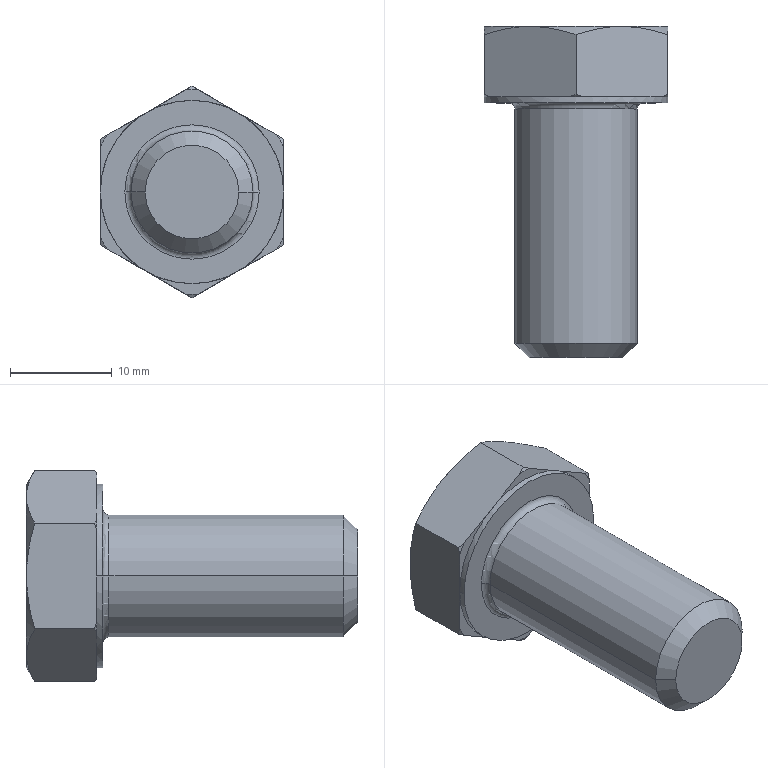Component | SolidWorks | GB_T5781-2000HexHeadBoltFullThreadCM12x25-2 | 1 solid | 35 faces | box 18 x 32.5 x 20.78 mm | volume 4879 mm3 | plane 15 | cone 14 | cylinder 4 | torus 2 | commonest cylinder face diameters 12 x2 18 x2 | material 3.6 Grade
STEP:
#1=CARTESIAN_POINT('',(0.5272,1.866,-3.022));
#2=VERTEX_POINT('',#1);
#3=CARTESIAN_POINT('',(0.05474,1.866,-3.022));
#4=VERTEX_POINT('',#3);
#5=CARTESIAN_POINT('',(0.291,1.866,-3.022));
#6=DIRECTION('',(0.,-1.,0.));
#7=DIRECTION('',(-1.,0.,0.));
#8=AXIS2_PLACEMENT_3D('',#5,#6,#7);
#9=CIRCLE('',#8,0.2362);
#10=EDGE_CURVE('',#2,#4,#9,.T.);
#11=ORIENTED_EDGE('',*,*,#10,.F.);
#12=CARTESIAN_POINT('',(0.5508,1.89,-3.022));
#13=VERTEX_POINT('',#12);
#14=CARTESIAN_POINT('',(0.5508,1.866,-3.022));
#15=DIRECTION('',(-0.,-0.,-1.));
#16=DIRECTION('',(-1.,0.,0.));
#17=AXIS2_PLACEMENT_3D('',#14,#15,#16);
#18=CIRCLE('',#17,0.02362);
#19=EDGE_CURVE('',#2,#13,#18,.T.);
#20=ORIENTED_EDGE('',*,*,#19,.T.);
#21=CARTESIAN_POINT('',(0.03111,1.89,-3.022));
#22=VERTEX_POINT('',#21);
#23=CARTESIAN_POINT('',(0.291,1.89,-3.022));
#24=DIRECTION('',(-0.,1.,-0.));
#25=DIRECTION('',(-1.,0.,0.));
#26=AXIS2_PLACEMENT_3D('',#23,#24,#25);
#27=CIRCLE('',#26,0.2598);
#28=EDGE_CURVE('',#22,#13,#27,.T.);
#29=ORIENTED_EDGE('',*,*,#28,.F.);
#30=CARTESIAN_POINT('',(0.03111,1.866,-3.022));
#31=DIRECTION('',(0.,0.,1.));
#32=DIRECTION('',(1.,0.,0.));
#33=AXIS2_PLACEMENT_3D('',#30,#31,#32);
#34=CIRCLE('',#33,0.02362);
#35=EDGE_CURVE('',#4,#22,#34,.T.);
#36=ORIENTED_EDGE('',*,*,#35,.F.);
#37=EDGE_LOOP('',(#11,#20,#29,#36));
#38=FACE_OUTER_BOUND('',#37,.T.);
#39=CARTESIAN_POINT('',(0.291,1.866,-3.022));
#40=DIRECTION('',(0.,-1.,0.));
#41=DIRECTION('',(-1.,-0.,0.));
#42=AXIS2_PLACEMENT_3D('',#39,#40,#41);
#43=TOROIDAL_SURFACE('',#42,0.2598,0.02362);
#44=ADVANCED_FACE('',(#38),#43,.F.);
#45=CARTESIAN_POINT('',(0.1099,0.9055,-3.022));
#46=VERTEX_POINT('',#45);
#47=CARTESIAN_POINT('',(0.4721,0.9055,-3.022));
#48=VERTEX_POINT('',#47);
#49=CARTESIAN_POINT('',(0.291,0.9055,-3.022));
#50=DIRECTION('',(0.,-1.,0.));
#51=DIRECTION('',(1.,0.,-0.));
#52=AXIS2_PLACEMENT_3D('',#49,#50,#51);
#53=CIRCLE('',#52,0.1811);
#54=EDGE_CURVE('',#46,#48,#53,.T.);
#55=ORIENTED_EDGE('',*,*,#54,.F.);
#56=CARTESIAN_POINT('',(0.05474,0.9606,-3.022));
#57=VERTEX_POINT('',#56);
#58=CARTESIAN_POINT('',(0.05474,0.9606,-3.022));
#59=DIRECTION('',(-0.7071,0.7071,0.));
#60=VECTOR('',#59,39.37);
#61=LINE('',#58,#60);
#62=EDGE_CURVE('',#46,#57,#61,.T.);
#63=ORIENTED_EDGE('',*,*,#62,.T.);
#64=CARTESIAN_POINT('',(0.5272,0.9606,-3.022));
#65=VERTEX_POINT('',#64);
#66=CARTESIAN_POINT('',(0.291,0.9606,-3.022));
#67=DIRECTION('',(-0.,1.,-0.));
#68=DIRECTION('',(1.,0.,-0.));
#69=AXIS2_PLACEMENT_3D('',#66,#67,#68);
#70=CIRCLE('',#69,0.2362);
#71=EDGE_CURVE('',#65,#57,#70,.T.);
#72=ORIENTED_EDGE('',*,*,#71,.F.);
#73=CARTESIAN_POINT('',(0.5272,0.9606,-3.022));
#74=DIRECTION('',(0.7071,0.7071,-0.));
#75=VECTOR('',#74,39.37);
#76=LINE('',#73,#75);
#77=EDGE_CURVE('',#48,#65,#76,.T.);
#78=ORIENTED_EDGE('',*,*,#77,.F.);
#79=EDGE_LOOP('',(#55,#63,#72,#78));
#80=FACE_OUTER_BOUND('',#79,.T.);
#81=CARTESIAN_POINT('',(0.291,0.9606,-3.022));
#82=DIRECTION('',(-0.,1.,-0.));
#83=DIRECTION('',(1.,0.,-0.));
#84=AXIS2_PLACEMENT_3D('',#81,#82,#83);
#85=CONICAL_SURFACE('',#84,0.2362,0.7854);
#86=ADVANCED_FACE('',(#80),#85,.T.);
#87=ORIENTED_EDGE('',*,*,#71,.T.);
#88=CARTESIAN_POINT('',(0.05474,2.185,-3.022));
#89=DIRECTION('',(-0.,1.,-0.));
#90=VECTOR('',#89,39.37);
#91=LINE('',#88,#90);
#92=EDGE_CURVE('',#57,#4,#91,.T.);
#93=ORIENTED_EDGE('',*,*,#92,.T.);
#94=CARTESIAN_POINT('',(0.291,1.866,-3.022));
#95=DIRECTION('',(0.,-1.,0.));
#96=DIRECTION('',(-1.,0.,0.));
#97=AXIS2_PLACEMENT_3D('',#94,#95,#96);
#98=CIRCLE('',#97,0.2362);
#99=EDGE_CURVE('',#4,#2,#98,.T.);
#100=ORIENTED_EDGE('',*,*,#99,.T.);
#101=CARTESIAN_POINT('',(0.5272,2.185,-3.022));
#102=DIRECTION('',(-0.,1.,-0.));
#103=VECTOR('',#102,39.37);
#104=LINE('',#101,#103);
#105=EDGE_CURVE('',#65,#2,#104,.T.);
#106=ORIENTED_EDGE('',*,*,#105,.F.);
#107=EDGE_LOOP('',(#87,#93,#100,#106));
#108=FACE_OUTER_BOUND('',#107,.T.);
#109=CARTESIAN_POINT('',(0.291,2.185,-3.022));
#110=DIRECTION('',(-0.,1.,-0.));
#111=DIRECTION('',(1.,0.,-0.));
#112=AXIS2_PLACEMENT_3D('',#109,#110,#111);
#113=CYLINDRICAL_SURFACE('',#112,0.2362);
#114=ADVANCED_FACE('',(#108),#113,.T.);
#115=CARTESIAN_POINT('',(-0.06337,1.89,-3.022));
#116=VERTEX_POINT('',#115);
#117=CARTESIAN_POINT('',(0.6453,1.89,-3.022));
#118=VERTEX_POINT('',#117);
#119=CARTESIAN_POINT('',(0.291,1.89,-3.022));
#120=DIRECTION('',(0.,-1.,0.));
#121=DIRECTION('',(-1.,0.,0.));
#122=AXIS2_PLACEMENT_3D('',#119,#120,#121);
#123=CIRCLE('',#122,0.3543);
#124=EDGE_CURVE('',#116,#118,#123,.T.);
#125=ORIENTED_EDGE('',*,*,#124,.F.);
#126=CARTESIAN_POINT('',(-0.06337,1.913,-3.022));
#127=VERTEX_POINT('',#126);
#128=CARTESIAN_POINT('',(-0.06337,2.185,-3.022));
#129=DIRECTION('',(-0.,1.,-0.));
#130=VECTOR('',#129,39.37);
#131=LINE('',#128,#130);
#132=EDGE_CURVE('',#116,#127,#131,.T.);
#133=ORIENTED_EDGE('',*,*,#132,.T.);
#134=CARTESIAN_POINT('',(0.1138,1.913,-3.329));
#135=VERTEX_POINT('',#134);
#136=CARTESIAN_POINT('',(0.291,1.913,-3.022));
#137=DIRECTION('',(-0.,1.,-0.));
#138=DIRECTION('',(1.,0.,-0.));
#139=AXIS2_PLACEMENT_3D('',#136,#137,#138);
#140=CIRCLE('',#139,0.3543);
#141=EDGE_CURVE('',#135,#127,#140,.T.);
#142=ORIENTED_EDGE('',*,*,#141,.F.);
#143=CARTESIAN_POINT('',(0.4681,1.913,-3.329));
#144=VERTEX_POINT('',#143);
#145=CARTESIAN_POINT('',(0.291,1.913,-3.022));
#146=DIRECTION('',(-0.,1.,-0.));
#147=DIRECTION('',(1.,0.,-0.));
#148=AXIS2_PLACEMENT_3D('',#145,#146,#147);
#149=CIRCLE('',#148,0.3543);
#150=EDGE_CURVE('',#144,#135,#149,.T.);
#151=ORIENTED_EDGE('',*,*,#150,.F.);
#152=CARTESIAN_POINT('',(0.6453,1.913,-3.022));
#153=VERTEX_POINT('',#152);
#154=CARTESIAN_POINT('',(0.291,1.913,-3.022));
#155=DIRECTION('',(-0.,1.,-0.));
#156=DIRECTION('',(1.,0.,-0.));
#157=AXIS2_PLACEMENT_3D('',#154,#155,#156);
#158=CIRCLE('',#157,0.3543);
#159=EDGE_CURVE('',#153,#144,#158,.T.);
#160=ORIENTED_EDGE('',*,*,#159,.F.);
#161=CARTESIAN_POINT('',(0.6453,2.185,-3.022));
#162=DIRECTION('',(-0.,1.,-0.));
#163=VECTOR('',#162,39.37);
#164=LINE('',#161,#163);
#165=EDGE_CURVE('',#118,#153,#164,.T.);
#166=ORIENTED_EDGE('',*,*,#165,.F.);
#167=EDGE_LOOP('',(#125,#133,#142,#151,#160,#166));
#168=FACE_OUTER_BOUND('',#167,.T.);
#169=CARTESIAN_POINT('',(0.291,2.185,-3.022));
#170=DIRECTION('',(-0.,1.,-0.));
#171=DIRECTION('',(1.,0.,-0.));
#172=AXIS2_PLACEMENT_3D('',#169,#170,#171);
#173=CYLINDRICAL_SURFACE('',#172,0.3543);
#174=ADVANCED_FACE('',(#168),#173,.T.);
#175=CARTESIAN_POINT('',(-0.03787,1.913,-3.241));
#176=VERTEX_POINT('',#175);
#177=CARTESIAN_POINT('',(-0.06337,1.913,-3.227));
#178=DIRECTION('',(0.866,0.,-0.5));
#179=VECTOR('',#178,39.37);
#180=LINE('',#177,#179);
#181=EDGE_CURVE('',#176,#135,#180,.T.);
#182=ORIENTED_EDGE('',*,*,#181,.F.);
#183=CARTESIAN_POINT('',(-0.06337,1.921,-3.227));
#184=VERTEX_POINT('',#183);
#185=CARTESIAN_POINT('',(-0.06337,1.921,-3.227));
#186=CARTESIAN_POINT('',(-0.05489,1.919,-3.232));
#187=CARTESIAN_POINT('',(-0.04639,1.916,-3.237));
#188=CARTESIAN_POINT('',(-0.03787,1.913,-3.241));
#189=B_SPLINE_CURVE_WITH_KNOTS('',3,(#185,#186,#187,#188),.UNSPECIFIED.,.F.,.F.,(4,4),(0.00000024,0.0007696),.UNSPECIFIED.);
#190=EDGE_CURVE('',#184,#176,#189,.T.);
#191=ORIENTED_EDGE('',*,*,#190,.F.);
#192=CARTESIAN_POINT('',(-0.06337,2.153,-3.227));
#193=VERTEX_POINT('',#192);
#194=CARTESIAN_POINT('',(-0.06337,1.89,-3.227));
#195=DIRECTION('',(-0.,1.,-0.));
#196=VECTOR('',#195,39.37);
#197=LINE('',#194,#196);
#198=EDGE_CURVE('',#184,#193,#197,.T.);
#199=ORIENTED_EDGE('',*,*,#198,.T.);
#200=CARTESIAN_POINT('',(0.1138,2.185,-3.329));
#201=VERTEX_POINT('',#200);
#202=CARTESIAN_POINT('',(0.1138,2.185,-3.329));
#203=CARTESIAN_POINT('',(0.09876,2.185,-3.32));
#204=CARTESIAN_POINT('',(0.08365,2.184,-3.312));
#205=CARTESIAN_POINT('',(0.05378,2.181,-3.294));
#206=CARTESIAN_POINT('',(0.03894,2.179,-3.286));
#207=CARTESIAN_POINT('',(-0.005313,2.171,-3.26));
#208=CARTESIAN_POINT('',(-0.03446,2.163,-3.243));
#209=CARTESIAN_POINT('',(-0.06337,2.153,-3.227));
#210=B_SPLINE_CURVE_WITH_KNOTS('',3,(#202,#203,#204,#205,#206,#207,#208,#209),.UNSPECIFIED.,.F.,.F.,(4,2,2,4),(0.005258,0.006567,0.007877,0.0105),.UNSPECIFIED.);
#211=EDGE_CURVE('',#201,#193,#210,.T.);
#212=ORIENTED_EDGE('',*,*,#211,.F.);
#213=CARTESIAN_POINT('',(0.291,2.153,-3.431));
#214=VERTEX_POINT('',#213);
#215=CARTESIAN_POINT('',(0.291,2.153,-3.431));
#216=CARTESIAN_POINT('',(0.262,2.163,-3.415));
#217=CARTESIAN_POINT('',(0.2328,2.171,-3.398));
#218=CARTESIAN_POINT('',(0.1738,2.182,-3.364));
#219=CARTESIAN_POINT('',(0.144,2.185,-3.346));
#220=CARTESIAN_POINT('',(0.1138,2.185,-3.329));
#221=B_SPLINE_CURVE_WITH_KNOTS('',3,(#215,#216,#217,#218,#219,#220),.UNSPECIFIED.,.F.,.F.,(4,2,4),(0.00000024,0.002629,0.005258),.UNSPECIFIED.);
#222=EDGE_CURVE('',#214,#201,#221,.T.);
#223=ORIENTED_EDGE('',*,*,#222,.F.);
#224=CARTESIAN_POINT('',(0.291,1.921,-3.431));
#225=VERTEX_POINT('',#224);
#226=CARTESIAN_POINT('',(0.291,1.89,-3.431));
#227=DIRECTION('',(-0.,1.,-0.));
#228=VECTOR('',#227,39.37);
#229=LINE('',#226,#228);
#230=EDGE_CURVE('',#225,#214,#229,.T.);
#231=ORIENTED_EDGE('',*,*,#230,.F.);
#232=CARTESIAN_POINT('',(0.2655,1.913,-3.417));
#233=VERTEX_POINT('',#232);
#234=CARTESIAN_POINT('',(0.2655,1.913,-3.417));
#235=CARTESIAN_POINT('',(0.274,1.916,-3.421));
#236=CARTESIAN_POINT('',(0.2825,1.919,-3.426));
#237=CARTESIAN_POINT('',(0.291,1.921,-3.431));
#238=B_SPLINE_CURVE_WITH_KNOTS('',3,(#234,#235,#236,#237),.UNSPECIFIED.,.F.,.F.,(4,4),(0.009728,0.0105),.UNSPECIFIED.);
#239=EDGE_CURVE('',#233,#225,#238,.T.);
#240=ORIENTED_EDGE('',*,*,#239,.F.);
#241=CARTESIAN_POINT('',(-0.06337,1.913,-3.227));
#242=DIRECTION('',(0.866,0.,-0.5));
#243=VECTOR('',#242,39.37);
#244=LINE('',#241,#243);
#245=EDGE_CURVE('',#135,#233,#244,.T.);
#246=ORIENTED_EDGE('',*,*,#245,.F.);
#247=EDGE_LOOP('',(#182,#191,#199,#212,#223,#231,#240,#246));
#248=FACE_OUTER_BOUND('',#247,.T.);
#249=CARTESIAN_POINT('',(-0.06337,1.89,-3.227));
#250=DIRECTION('',(0.5,0.,0.866));
#251=DIRECTION('',(-0.866,-0.,0.5));
#252=AXIS2_PLACEMENT_3D('',#249,#250,#251);
#253=PLANE('',#252);
#254=ADVANCED_FACE('',(#248),#253,.F.);
#255=CARTESIAN_POINT('',(0.3165,1.913,-3.417));
#256=VERTEX_POINT('',#255);
#257=CARTESIAN_POINT('',(0.291,1.913,-3.431));
#258=DIRECTION('',(0.866,0.,0.5));
#259=VECTOR('',#258,39.37);
#260=LINE('',#257,#259);
#261=EDGE_CURVE('',#256,#144,#260,.T.);
#262=ORIENTED_EDGE('',*,*,#261,.F.);
#263=CARTESIAN_POINT('',(0.291,1.921,-3.431));
#264=CARTESIAN_POINT('',(0.2994,1.919,-3.426));
#265=CARTESIAN_POINT('',(0.3079,1.916,-3.421));
#266=CARTESIAN_POINT('',(0.3165,1.913,-3.417));
#267=B_SPLINE_CURVE_WITH_KNOTS('',3,(#263,#264,#265,#266),.UNSPECIFIED.,.F.,.F.,(4,4),(0.00000024,0.0007696),.UNSPECIFIED.);
#268=EDGE_CURVE('',#225,#256,#267,.T.);
#269=ORIENTED_EDGE('',*,*,#268,.F.);
#270=ORIENTED_EDGE('',*,*,#230,.T.);
#271=CARTESIAN_POINT('',(0.4681,2.185,-3.329));
#272=VERTEX_POINT('',#271);
#273=CARTESIAN_POINT('',(0.4681,2.185,-3.329));
#274=CARTESIAN_POINT('',(0.4531,2.185,-3.338));
#275=CARTESIAN_POINT('',(0.438,2.184,-3.346));
#276=CARTESIAN_POINT('',(0.4081,2.181,-3.364));
#277=CARTESIAN_POINT('',(0.3933,2.179,-3.372));
#278=CARTESIAN_POINT('',(0.349,2.171,-3.398));
#279=CARTESIAN_POINT('',(0.3199,2.163,-3.415));
#280=CARTESIAN_POINT('',(0.291,2.153,-3.431));
#281=B_SPLINE_CURVE_WITH_KNOTS('',3,(#273,#274,#275,#276,#277,#278,#279,#280),.UNSPECIFIED.,.F.,.F.,(4,2,2,4),(0.005258,0.006567,0.007877,0.0105),.UNSPECIFIED.);
#282=EDGE_CURVE('',#272,#214,#281,.T.);
#283=ORIENTED_EDGE('',*,*,#282,.F.);
#284=CARTESIAN_POINT('',(0.6453,2.153,-3.227));
#285=VERTEX_POINT('',#284);
#286=CARTESIAN_POINT('',(0.6453,2.153,-3.227));
#287=CARTESIAN_POINT('',(0.6163,2.163,-3.243));
#288=CARTESIAN_POINT('',(0.5871,2.171,-3.26));
#289=CARTESIAN_POINT('',(0.5281,2.182,-3.294));
#290=CARTESIAN_POINT('',(0.4983,2.185,-3.312));
#291=CARTESIAN_POINT('',(0.4681,2.185,-3.329));
#292=B_SPLINE_CURVE_WITH_KNOTS('',3,(#286,#287,#288,#289,#290,#291),.UNSPECIFIED.,.F.,.F.,(4,2,4),(0.00000024,0.002629,0.005258),.UNSPECIFIED.);
#293=EDGE_CURVE('',#285,#272,#292,.T.);
#294=ORIENTED_EDGE('',*,*,#293,.F.);
#295=CARTESIAN_POINT('',(0.6453,1.921,-3.227));
#296=VERTEX_POINT('',#295);
#297=CARTESIAN_POINT('',(0.6453,1.89,-3.227));
#298=DIRECTION('',(-0.,1.,-0.));
#299=VECTOR('',#298,39.37);
#300=LINE('',#297,#299);
#301=EDGE_CURVE('',#296,#285,#300,.T.);
#302=ORIENTED_EDGE('',*,*,#301,.F.);
#303=CARTESIAN_POINT('',(0.6198,1.913,-3.241));
#304=VERTEX_POINT('',#303);
#305=CARTESIAN_POINT('',(0.6198,1.913,-3.241));
#306=CARTESIAN_POINT('',(0.6283,1.916,-3.237));
#307=CARTESIAN_POINT('',(0.6368,1.919,-3.232));
#308=CARTESIAN_POINT('',(0.6453,1.921,-3.227));
#309=B_SPLINE_CURVE_WITH_KNOTS('',3,(#305,#306,#307,#308),.UNSPECIFIED.,.F.,.F.,(4,4),(0.009728,0.0105),.UNSPECIFIED.);
#310=EDGE_CURVE('',#304,#296,#309,.T.);
#311=ORIENTED_EDGE('',*,*,#310,.F.);
#312=CARTESIAN_POINT('',(0.291,1.913,-3.431));
#313=DIRECTION('',(0.866,0.,0.5));
#314=VECTOR('',#313,39.37);
#315=LINE('',#312,#314);
#316=EDGE_CURVE('',#144,#304,#315,.T.);
#317=ORIENTED_EDGE('',*,*,#316,.F.);
#318=EDGE_LOOP('',(#262,#269,#270,#283,#294,#302,#311,#317));
#319=FACE_OUTER_BOUND('',#318,.T.);
#320=CARTESIAN_POINT('',(0.291,1.89,-3.431));
#321=DIRECTION('',(-0.5,0.,0.866));
#322=DIRECTION('',(-0.866,-0.,-0.5));
#323=AXIS2_PLACEMENT_3D('',#320,#321,#322);
#324=PLANE('',#323);
#325=ADVANCED_FACE('',(#319),#324,.F.);
#326=CARTESIAN_POINT('',(0.6453,1.913,-3.197));
#327=VERTEX_POINT('',#326);
#328=CARTESIAN_POINT('',(0.6453,1.913,-3.227));
#329=DIRECTION('',(0.,0.,1.));
#330=VECTOR('',#329,39.37);
#331=LINE('',#328,#330);
#332=EDGE_CURVE('',#327,#153,#331,.T.);
#333=ORIENTED_EDGE('',*,*,#332,.F.);
#334=CARTESIAN_POINT('',(0.6453,1.921,-3.227));
#335=CARTESIAN_POINT('',(0.6453,1.919,-3.217));
#336=CARTESIAN_POINT('',(0.6453,1.916,-3.207));
#337=CARTESIAN_POINT('',(0.6453,1.913,-3.197));
#338=B_SPLINE_CURVE_WITH_KNOTS('',3,(#334,#335,#336,#337),.UNSPECIFIED.,.F.,.F.,(4,4),(0.02519,0.02597),.UNSPECIFIED.);
#339=EDGE_CURVE('',#296,#327,#338,.T.);
#340=ORIENTED_EDGE('',*,*,#339,.F.);
#341=ORIENTED_EDGE('',*,*,#301,.T.);
#342=CARTESIAN_POINT('',(0.6453,2.185,-3.022));
#343=VERTEX_POINT('',#342);
#344=CARTESIAN_POINT('',(0.6453,2.185,-3.022));
#345=CARTESIAN_POINT('',(0.6453,2.185,-3.039));
#346=CARTESIAN_POINT('',(0.6453,2.184,-3.057));
#347=CARTESIAN_POINT('',(0.6453,2.181,-3.092));
#348=CARTESIAN_POINT('',(0.6453,2.179,-3.109));
#349=CARTESIAN_POINT('',(0.6453,2.171,-3.16));
#350=CARTESIAN_POINT('',(0.6453,2.163,-3.194));
#351=CARTESIAN_POINT('',(0.6453,2.153,-3.227));
#352=B_SPLINE_CURVE_WITH_KNOTS('',3,(#344,#345,#346,#347,#348,#349,#350,#351),.UNSPECIFIED.,.F.,.F.,(4,2,2,4),(0.01498,0.0163,0.01761,0.02025),.UNSPECIFIED.);
#353=EDGE_CURVE('',#343,#285,#352,.T.);
#354=ORIENTED_EDGE('',*,*,#353,.F.);
#355=CARTESIAN_POINT('',(0.6453,2.153,-2.818));
#356=VERTEX_POINT('',#355);
#357=CARTESIAN_POINT('',(0.6453,2.153,-2.818));
#358=CARTESIAN_POINT('',(0.6453,2.163,-2.851));
#359=CARTESIAN_POINT('',(0.6453,2.171,-2.885));
#360=CARTESIAN_POINT('',(0.6453,2.182,-2.953));
#361=CARTESIAN_POINT('',(0.6453,2.185,-2.988));
#362=CARTESIAN_POINT('',(0.6453,2.185,-3.022));
#363=B_SPLINE_CURVE_WITH_KNOTS('',3,(#357,#358,#359,#360,#361,#362),.UNSPECIFIED.,.F.,.F.,(4,2,4),(0.00972,0.01235,0.01498),.UNSPECIFIED.);
#364=EDGE_CURVE('',#356,#343,#363,.T.);
#365=ORIENTED_EDGE('',*,*,#364,.F.);
#366=CARTESIAN_POINT('',(0.6453,1.921,-2.818));
#367=VERTEX_POINT('',#366);
#368=CARTESIAN_POINT('',(0.6453,1.89,-2.818));
#369=DIRECTION('',(-0.,1.,-0.));
#370=VECTOR('',#369,39.37);
#371=LINE('',#368,#370);
#372=EDGE_CURVE('',#367,#356,#371,.T.);
#373=ORIENTED_EDGE('',*,*,#372,.F.);
#374=CARTESIAN_POINT('',(0.6453,1.913,-2.847));
#375=VERTEX_POINT('',#374);
#376=CARTESIAN_POINT('',(0.6453,1.913,-2.847));
#377=CARTESIAN_POINT('',(0.6453,1.916,-2.837));
#378=CARTESIAN_POINT('',(0.6453,1.919,-2.827));
#379=CARTESIAN_POINT('',(0.6453,1.921,-2.818));
#380=B_SPLINE_CURVE_WITH_KNOTS('',3,(#376,#377,#378,#379),.UNSPECIFIED.,.F.,.F.,(4,4),(0.03494,0.03571),.UNSPECIFIED.);
#381=EDGE_CURVE('',#375,#367,#380,.T.);
#382=ORIENTED_EDGE('',*,*,#381,.F.);
#383=CARTESIAN_POINT('',(0.6453,1.913,-3.227));
#384=DIRECTION('',(0.,0.,1.));
#385=VECTOR('',#384,39.37);
#386=LINE('',#383,#385);
#387=EDGE_CURVE('',#153,#375,#386,.T.);
#388=ORIENTED_EDGE('',*,*,#387,.F.);
#389=EDGE_LOOP('',(#333,#340,#341,#354,#365,#373,#382,#388));
#390=FACE_OUTER_BOUND('',#389,.T.);
#391=CARTESIAN_POINT('',(0.6453,1.89,-3.227));
#392=DIRECTION('',(-1.,-0.,0.));
#393=DIRECTION('',(-0.,-0.,-1.));
#394=AXIS2_PLACEMENT_3D('',#391,#392,#393);
#395=PLANE('',#394);
#396=ADVANCED_FACE('',(#390),#395,.F.);
#397=CARTESIAN_POINT('',(0.6198,1.913,-2.803));
#398=VERTEX_POINT('',#397);
#399=CARTESIAN_POINT('',(0.4681,1.913,-2.715));
#400=VERTEX_POINT('',#399);
#401=CARTESIAN_POINT('',(0.291,1.913,-2.613));
#402=DIRECTION('',(-0.866,-0.,0.5));
#403=VECTOR('',#402,39.37);
#404=LINE('',#401,#403);
#405=EDGE_CURVE('',#398,#400,#404,.T.);
#406=ORIENTED_EDGE('',*,*,#405,.F.);
#407=CARTESIAN_POINT('',(0.6453,1.921,-2.818));
#408=CARTESIAN_POINT('',(0.6368,1.919,-2.813));
#409=CARTESIAN_POINT('',(0.6283,1.916,-2.808));
#410=CARTESIAN_POINT('',(0.6198,1.913,-2.803));
#411=B_SPLINE_CURVE_WITH_KNOTS('',3,(#407,#408,#409,#410),.UNSPECIFIED.,.F.,.F.,(4,4),(0.00000024,0.0007696),.UNSPECIFIED.);
#412=EDGE_CURVE('',#367,#398,#411,.T.);
#413=ORIENTED_EDGE('',*,*,#412,.F.);
#414=ORIENTED_EDGE('',*,*,#372,.T.);
#415=CARTESIAN_POINT('',(0.4681,2.185,-2.715));
#416=VERTEX_POINT('',#415);
#417=CARTESIAN_POINT('',(0.4681,2.185,-2.715));
#418=CARTESIAN_POINT('',(0.4832,2.185,-2.724));
#419=CARTESIAN_POINT('',(0.4983,2.184,-2.733));
#420=CARTESIAN_POINT('',(0.5281,2.181,-2.75));
#421=CARTESIAN_POINT('',(0.543,2.179,-2.759));
#422=CARTESIAN_POINT('',(0.5872,2.171,-2.784));
#423=CARTESIAN_POINT('',(0.6164,2.163,-2.801));
#424=CARTESIAN_POINT('',(0.6453,2.153,-2.818));
#425=B_SPLINE_CURVE_WITH_KNOTS('',3,(#417,#418,#419,#420,#421,#422,#423,#424),.UNSPECIFIED.,.F.,.F.,(4,2,2,4),(0.005258,0.006567,0.007877,0.0105),.UNSPECIFIED.);
#426=EDGE_CURVE('',#416,#356,#425,.T.);
#427=ORIENTED_EDGE('',*,*,#426,.F.);
#428=CARTESIAN_POINT('',(0.291,2.153,-2.613));
#429=VERTEX_POINT('',#428);
#430=CARTESIAN_POINT('',(0.291,2.153,-2.613));
#431=CARTESIAN_POINT('',(0.3199,2.163,-2.63));
#432=CARTESIAN_POINT('',(0.3491,2.171,-2.647));
#433=CARTESIAN_POINT('',(0.4081,2.182,-2.681));
#434=CARTESIAN_POINT('',(0.4379,2.185,-2.698));
#435=CARTESIAN_POINT('',(0.4681,2.185,-2.715));
#436=B_SPLINE_CURVE_WITH_KNOTS('',3,(#430,#431,#432,#433,#434,#435),.UNSPECIFIED.,.F.,.F.,(4,2,4),(0.00000024,0.002629,0.005258),.UNSPECIFIED.);
#437=EDGE_CURVE('',#429,#416,#436,.T.);
#438=ORIENTED_EDGE('',*,*,#437,.F.);
#439=CARTESIAN_POINT('',(0.291,1.921,-2.613));
#440=VERTEX_POINT('',#439);
#441=CARTESIAN_POINT('',(0.291,1.89,-2.613));
#442=DIRECTION('',(-0.,1.,-0.));
#443=VECTOR('',#442,39.37);
#444=LINE('',#441,#443);
#445=EDGE_CURVE('',#440,#429,#444,.T.);
#446=ORIENTED_EDGE('',*,*,#445,.F.);
#447=CARTESIAN_POINT('',(0.3165,1.913,-2.628));
#448=VERTEX_POINT('',#447);
#449=CARTESIAN_POINT('',(0.3165,1.913,-2.628));
#450=CARTESIAN_POINT('',(0.3079,1.916,-2.623));
#451=CARTESIAN_POINT('',(0.2994,1.919,-2.618));
#452=CARTESIAN_POINT('',(0.291,1.921,-2.613));
#453=B_SPLINE_CURVE_WITH_KNOTS('',3,(#449,#450,#451,#452),.UNSPECIFIED.,.F.,.F.,(4,4),(0.009728,0.0105),.UNSPECIFIED.);
#454=EDGE_CURVE('',#448,#440,#453,.T.);
#455=ORIENTED_EDGE('',*,*,#454,.F.);
#456=CARTESIAN_POINT('',(0.291,1.913,-2.613));
#457=DIRECTION('',(-0.866,-0.,0.5));
#458=VECTOR('',#457,39.37);
#459=LINE('',#456,#458);
#460=EDGE_CURVE('',#400,#448,#459,.T.);
#461=ORIENTED_EDGE('',*,*,#460,.F.);
#462=EDGE_LOOP('',(#406,#413,#414,#427,#438,#446,#455,#461));
#463=FACE_OUTER_BOUND('',#462,.T.);
#464=CARTESIAN_POINT('',(0.291,1.89,-2.613));
#465=DIRECTION('',(-0.5,-0.,-0.866));
#466=DIRECTION('',(0.866,0.,-0.5));
#467=AXIS2_PLACEMENT_3D('',#464,#465,#466);
#468=PLANE('',#467);
#469=ADVANCED_FACE('',(#463),#468,.F.);
#470=CARTESIAN_POINT('',(0.2655,1.913,-2.628));
#471=VERTEX_POINT('',#470);
#472=CARTESIAN_POINT('',(0.1138,1.913,-2.715));
#473=VERTEX_POINT('',#472);
#474=CARTESIAN_POINT('',(-0.06337,1.913,-2.818));
#475=DIRECTION('',(-0.866,-0.,-0.5));
#476=VECTOR('',#475,39.37);
#477=LINE('',#474,#476);
#478=EDGE_CURVE('',#471,#473,#477,.T.);
#479=ORIENTED_EDGE('',*,*,#478,.F.);
#480=CARTESIAN_POINT('',(0.291,1.921,-2.613));
#481=CARTESIAN_POINT('',(0.2825,1.919,-2.618));
#482=CARTESIAN_POINT('',(0.274,1.916,-2.623));
#483=CARTESIAN_POINT('',(0.2655,1.913,-2.628));
#484=B_SPLINE_CURVE_WITH_KNOTS('',3,(#480,#481,#482,#483),.UNSPECIFIED.,.F.,.F.,(4,4),(0.00000024,0.0007696),.UNSPECIFIED.);
#485=EDGE_CURVE('',#440,#471,#484,.T.);
#486=ORIENTED_EDGE('',*,*,#485,.F.);
#487=ORIENTED_EDGE('',*,*,#445,.T.);
#488=CARTESIAN_POINT('',(0.1138,2.185,-2.715));
#489=VERTEX_POINT('',#488);
#490=CARTESIAN_POINT('',(0.1138,2.185,-2.715));
#491=CARTESIAN_POINT('',(0.1288,2.185,-2.707));
#492=CARTESIAN_POINT('',(0.1439,2.184,-2.698));
#493=CARTESIAN_POINT('',(0.1738,2.181,-2.681));
#494=CARTESIAN_POINT('',(0.1886,2.179,-2.672));
#495=CARTESIAN_POINT('',(0.2329,2.171,-2.647));
#496=CARTESIAN_POINT('',(0.262,2.163,-2.63));
#497=CARTESIAN_POINT('',(0.291,2.153,-2.613));
#498=B_SPLINE_CURVE_WITH_KNOTS('',3,(#490,#491,#492,#493,#494,#495,#496,#497),.UNSPECIFIED.,.F.,.F.,(4,2,2,4),(0.005258,0.006567,0.007877,0.0105),.UNSPECIFIED.);
#499=EDGE_CURVE('',#489,#429,#498,.T.);
#500=ORIENTED_EDGE('',*,*,#499,.F.);
#501=CARTESIAN_POINT('',(-0.06337,2.153,-2.818));
#502=VERTEX_POINT('',#501);
#503=CARTESIAN_POINT('',(-0.06337,2.153,-2.818));
#504=CARTESIAN_POINT('',(-0.03439,2.163,-2.801));
#505=CARTESIAN_POINT('',(-0.005198,2.171,-2.784));
#506=CARTESIAN_POINT('',(0.0538,2.182,-2.75));
#507=CARTESIAN_POINT('',(0.08361,2.185,-2.733));
#508=CARTESIAN_POINT('',(0.1138,2.185,-2.715));
#509=B_SPLINE_CURVE_WITH_KNOTS('',3,(#503,#504,#505,#506,#507,#508),.UNSPECIFIED.,.F.,.F.,(4,2,4),(0.00000024,0.002629,0.005258),.UNSPECIFIED.);
#510=EDGE_CURVE('',#502,#489,#509,.T.);
#511=ORIENTED_EDGE('',*,*,#510,.F.);
#512=CARTESIAN_POINT('',(-0.06337,1.921,-2.818));
#513=VERTEX_POINT('',#512);
#514=CARTESIAN_POINT('',(-0.06337,1.89,-2.818));
#515=DIRECTION('',(-0.,1.,-0.));
#516=VECTOR('',#515,39.37);
#517=LINE('',#514,#516);
#518=EDGE_CURVE('',#513,#502,#517,.T.);
#519=ORIENTED_EDGE('',*,*,#518,.F.);
#520=CARTESIAN_POINT('',(-0.03787,1.913,-2.803));
#521=VERTEX_POINT('',#520);
#522=CARTESIAN_POINT('',(-0.03787,1.913,-2.803));
#523=CARTESIAN_POINT('',(-0.04639,1.916,-2.808));
#524=CARTESIAN_POINT('',(-0.05489,1.919,-2.813));
#525=CARTESIAN_POINT('',(-0.06337,1.921,-2.818));
#526=B_SPLINE_CURVE_WITH_KNOTS('',3,(#522,#523,#524,#525),.UNSPECIFIED.,.F.,.F.,(4,4),(0.009728,0.0105),.UNSPECIFIED.);
#527=EDGE_CURVE('',#521,#513,#526,.T.);
#528=ORIENTED_EDGE('',*,*,#527,.F.);
#529=CARTESIAN_POINT('',(-0.06337,1.913,-2.818));
#530=DIRECTION('',(-0.866,-0.,-0.5));
#531=VECTOR('',#530,39.37);
#532=LINE('',#529,#531);
#533=EDGE_CURVE('',#473,#521,#532,.T.);
#534=ORIENTED_EDGE('',*,*,#533,.F.);
#535=EDGE_LOOP('',(#479,#486,#487,#500,#511,#519,#528,#534));
#536=FACE_OUTER_BOUND('',#535,.T.);
#537=CARTESIAN_POINT('',(-0.06337,1.89,-2.818));
#538=DIRECTION('',(0.5,-0.,-0.866));
#539=DIRECTION('',(0.866,0.,0.5));
#540=AXIS2_PLACEMENT_3D('',#537,#538,#539);
#541=PLANE('',#540);
#542=ADVANCED_FACE('',(#536),#541,.F.);
#543=CARTESIAN_POINT('',(-0.06337,1.913,-2.847));
#544=VERTEX_POINT('',#543);
#545=CARTESIAN_POINT('',(-0.06337,1.913,-3.227));
#546=DIRECTION('',(-0.,-0.,-1.));
#547=VECTOR('',#546,39.37);
#548=LINE('',#545,#547);
#549=EDGE_CURVE('',#544,#127,#548,.T.);
#550=ORIENTED_EDGE('',*,*,#549,.F.);
#551=CARTESIAN_POINT('',(-0.06337,1.921,-2.818));
#552=CARTESIAN_POINT('',(-0.06337,1.919,-2.827));
#553=CARTESIAN_POINT('',(-0.06337,1.916,-2.837));
#554=CARTESIAN_POINT('',(-0.06337,1.913,-2.847));
#555=B_SPLINE_CURVE_WITH_KNOTS('',3,(#551,#552,#553,#554),.UNSPECIFIED.,.F.,.F.,(4,4),(0.00972,0.01049),.UNSPECIFIED.);
#556=EDGE_CURVE('',#513,#544,#555,.T.);
#557=ORIENTED_EDGE('',*,*,#556,.F.);
#558=ORIENTED_EDGE('',*,*,#518,.T.);
#559=CARTESIAN_POINT('',(-0.06337,2.185,-3.022));
#560=VERTEX_POINT('',#559);
#561=CARTESIAN_POINT('',(-0.06337,2.185,-3.022));
#562=CARTESIAN_POINT('',(-0.06337,2.185,-2.988));
#563=CARTESIAN_POINT('',(-0.06337,2.182,-2.953));
#564=CARTESIAN_POINT('',(-0.06337,2.171,-2.885));
#565=CARTESIAN_POINT('',(-0.06337,2.163,-2.851));
#566=CARTESIAN_POINT('',(-0.06337,2.153,-2.818));
#567=B_SPLINE_CURVE_WITH_KNOTS('',3,(#561,#562,#563,#564,#565,#566),.UNSPECIFIED.,.F.,.F.,(4,2,4),(0.03045,0.03308,0.03571),.UNSPECIFIED.);
#568=EDGE_CURVE('',#560,#502,#567,.T.);
#569=ORIENTED_EDGE('',*,*,#568,.F.);
#570=CARTESIAN_POINT('',(-0.06337,2.153,-3.227));
#571=CARTESIAN_POINT('',(-0.06337,2.163,-3.194));
#572=CARTESIAN_POINT('',(-0.06337,2.171,-3.16));
#573=CARTESIAN_POINT('',(-0.06337,2.179,-3.109));
#574=CARTESIAN_POINT('',(-0.06337,2.181,-3.092));
#575=CARTESIAN_POINT('',(-0.06337,2.184,-3.057));
#576=CARTESIAN_POINT('',(-0.06337,2.185,-3.039));
#577=CARTESIAN_POINT('',(-0.06337,2.185,-3.022));
#578=B_SPLINE_CURVE_WITH_KNOTS('',3,(#570,#571,#572,#573,#574,#575,#576,#577),.UNSPECIFIED.,.F.,.F.,(4,2,2,4),(0.02519,0.02782,0.02914,0.03045),.UNSPECIFIED.);
#579=EDGE_CURVE('',#193,#560,#578,.T.);
#580=ORIENTED_EDGE('',*,*,#579,.F.);
#581=ORIENTED_EDGE('',*,*,#198,.F.);
#582=CARTESIAN_POINT('',(-0.06337,1.913,-3.197));
#583=VERTEX_POINT('',#582);
#584=CARTESIAN_POINT('',(-0.06337,1.913,-3.197));
#585=CARTESIAN_POINT('',(-0.06337,1.916,-3.207));
#586=CARTESIAN_POINT('',(-0.06337,1.919,-3.217));
#587=CARTESIAN_POINT('',(-0.06337,1.921,-3.227));
#588=B_SPLINE_CURVE_WITH_KNOTS('',3,(#584,#585,#586,#587),.UNSPECIFIED.,.F.,.F.,(4,4),(0.01947,0.02025),.UNSPECIFIED.);
#589=EDGE_CURVE('',#583,#184,#588,.T.);
#590=ORIENTED_EDGE('',*,*,#589,.F.);
#591=CARTESIAN_POINT('',(-0.06337,1.913,-3.227));
#592=DIRECTION('',(-0.,-0.,-1.));
#593=VECTOR('',#592,39.37);
#594=LINE('',#591,#593);
#595=EDGE_CURVE('',#127,#583,#594,.T.);
#596=ORIENTED_EDGE('',*,*,#595,.F.);
#597=EDGE_LOOP('',(#550,#557,#558,#569,#580,#581,#590,#596));
#598=FACE_OUTER_BOUND('',#597,.T.);
#599=CARTESIAN_POINT('',(-0.06337,1.89,-3.227));
#600=DIRECTION('',(1.,0.,-0.));
#601=DIRECTION('',(0.,-1.,0.));
#602=AXIS2_PLACEMENT_3D('',#599,#600,#601);
#603=PLANE('',#602);
#604=ADVANCED_FACE('',(#598),#603,.F.);
#605=ORIENTED_EDGE('',*,*,#556,.T.);
#606=CARTESIAN_POINT('',(0.291,1.913,-3.022));
#607=DIRECTION('',(-0.,1.,-0.));
#608=DIRECTION('',(-1.,0.,0.));
#609=AXIS2_PLACEMENT_3D('',#606,#607,#608);
#610=CIRCLE('',#609,0.3952);
#611=EDGE_CURVE('',#544,#521,#610,.T.);
#612=ORIENTED_EDGE('',*,*,#611,.T.);
#613=ORIENTED_EDGE('',*,*,#527,.T.);
#614=EDGE_LOOP('',(#605,#612,#613));
#615=FACE_OUTER_BOUND('',#614,.T.);
#616=CARTESIAN_POINT('',(0.291,2.035,-3.022));
#617=DIRECTION('',(-0.,1.,-0.));
#618=DIRECTION('',(1.,0.,-0.));
#619=AXIS2_PLACEMENT_3D('',#616,#617,#618);
#620=CONICAL_SURFACE('',#619,0.606,1.047);
#621=ADVANCED_FACE('',(#615),#620,.T.);
#622=ORIENTED_EDGE('',*,*,#485,.T.);
#623=CARTESIAN_POINT('',(0.291,1.913,-3.022));
#624=DIRECTION('',(-0.,1.,-0.));
#625=DIRECTION('',(-1.,0.,0.));
#626=AXIS2_PLACEMENT_3D('',#623,#624,#625);
#627=CIRCLE('',#626,0.3952);
#628=EDGE_CURVE('',#471,#448,#627,.T.);
#629=ORIENTED_EDGE('',*,*,#628,.T.);
#630=ORIENTED_EDGE('',*,*,#454,.T.);
#631=EDGE_LOOP('',(#622,#629,#630));
#632=FACE_OUTER_BOUND('',#631,.T.);
#633=CARTESIAN_POINT('',(0.291,2.035,-3.022));
#634=DIRECTION('',(-0.,1.,-0.));
#635=DIRECTION('',(1.,0.,-0.));
#636=AXIS2_PLACEMENT_3D('',#633,#634,#635);
#637=CONICAL_SURFACE('',#636,0.606,1.047);
#638=ADVANCED_FACE('',(#632),#637,.T.);
#639=ORIENTED_EDGE('',*,*,#412,.T.);
#640=CARTESIAN_POINT('',(0.291,1.913,-3.022));
#641=DIRECTION('',(-0.,1.,-0.));
#642=DIRECTION('',(-1.,0.,0.));
#643=AXIS2_PLACEMENT_3D('',#640,#641,#642);
#644=CIRCLE('',#643,0.3952);
#645=EDGE_CURVE('',#398,#375,#644,.T.);
#646=ORIENTED_EDGE('',*,*,#645,.T.);
#647=ORIENTED_EDGE('',*,*,#381,.T.);
#648=EDGE_LOOP('',(#639,#646,#647));
#649=FACE_OUTER_BOUND('',#648,.T.);
#650=CARTESIAN_POINT('',(0.291,2.035,-3.022));
#651=DIRECTION('',(-0.,1.,-0.));
#652=DIRECTION('',(1.,0.,-0.));
#653=AXIS2_PLACEMENT_3D('',#650,#651,#652);
#654=CONICAL_SURFACE('',#653,0.606,1.047);
#655=ADVANCED_FACE('',(#649),#654,.T.);
#656=ORIENTED_EDGE('',*,*,#339,.T.);
#657=CARTESIAN_POINT('',(0.291,1.913,-3.022));
#658=DIRECTION('',(-0.,1.,-0.));
#659=DIRECTION('',(-1.,0.,0.));
#660=AXIS2_PLACEMENT_3D('',#657,#658,#659);
#661=CIRCLE('',#660,0.3952);
#662=EDGE_CURVE('',#327,#304,#661,.T.);
#663=ORIENTED_EDGE('',*,*,#662,.T.);
#664=ORIENTED_EDGE('',*,*,#310,.T.);
#665=EDGE_LOOP('',(#656,#663,#664));
#666=FACE_OUTER_BOUND('',#665,.T.);
#667=CARTESIAN_POINT('',(0.291,2.035,-3.022));
#668=DIRECTION('',(-0.,1.,-0.));
#669=DIRECTION('',(1.,0.,-0.));
#670=AXIS2_PLACEMENT_3D('',#667,#668,#669);
#671=CONICAL_SURFACE('',#670,0.606,1.047);
#672=ADVANCED_FACE('',(#666),#671,.T.);
#673=ORIENTED_EDGE('',*,*,#268,.T.);
#674=CARTESIAN_POINT('',(0.291,1.913,-3.022));
#675=DIRECTION('',(-0.,1.,-0.));
#676=DIRECTION('',(-1.,0.,0.));
#677=AXIS2_PLACEMENT_3D('',#674,#675,#676);
#678=CIRCLE('',#677,0.3952);
#679=EDGE_CURVE('',#256,#233,#678,.T.);
#680=ORIENTED_EDGE('',*,*,#679,.T.);
#681=ORIENTED_EDGE('',*,*,#239,.T.);
#682=EDGE_LOOP('',(#673,#680,#681));
#683=FACE_OUTER_BOUND('',#682,.T.);
#684=CARTESIAN_POINT('',(0.291,2.035,-3.022));
#685=DIRECTION('',(-0.,1.,-0.));
#686=DIRECTION('',(1.,0.,-0.));
#687=AXIS2_PLACEMENT_3D('',#684,#685,#686);
#688=CONICAL_SURFACE('',#687,0.606,1.047);
#689=ADVANCED_FACE('',(#683),#688,.T.);
#690=ORIENTED_EDGE('',*,*,#190,.T.);
#691=CARTESIAN_POINT('',(0.291,1.913,-3.022));
#692=DIRECTION('',(-0.,1.,-0.));
#693=DIRECTION('',(-1.,0.,-0.));
#694=AXIS2_PLACEMENT_3D('',#691,#692,#693);
#695=CIRCLE('',#694,0.3952);
#696=EDGE_CURVE('',#176,#583,#695,.T.);
#697=ORIENTED_EDGE('',*,*,#696,.T.);
#698=ORIENTED_EDGE('',*,*,#589,.T.);
#699=EDGE_LOOP('',(#690,#697,#698));
#700=FACE_OUTER_BOUND('',#699,.T.);
#701=CARTESIAN_POINT('',(0.291,2.035,-3.022));
#702=DIRECTION('',(-0.,1.,-0.));
#703=DIRECTION('',(1.,0.,-0.));
#704=AXIS2_PLACEMENT_3D('',#701,#702,#703);
#705=CONICAL_SURFACE('',#704,0.606,1.047);
#706=ADVANCED_FACE('',(#700),#705,.T.);
#707=ORIENTED_EDGE('',*,*,#510,.T.);
#708=CARTESIAN_POINT('',(0.291,2.185,-3.022));
#709=DIRECTION('',(0.,-1.,0.));
#710=DIRECTION('',(-1.,0.,0.));
#711=AXIS2_PLACEMENT_3D('',#708,#709,#710);
#712=CIRCLE('',#711,0.3543);
#713=EDGE_CURVE('',#489,#560,#712,.T.);
#714=ORIENTED_EDGE('',*,*,#713,.T.);
#715=ORIENTED_EDGE('',*,*,#568,.T.);
#716=EDGE_LOOP('',(#707,#714,#715));
#717=FACE_OUTER_BOUND('',#716,.T.);
#718=CARTESIAN_POINT('',(0.291,2.185,-3.022));
#719=DIRECTION('',(0.,-1.,0.));
#720=DIRECTION('',(-1.,0.,0.));
#721=AXIS2_PLACEMENT_3D('',#718,#719,#720);
#722=CONICAL_SURFACE('',#721,0.3543,1.047);
#723=ADVANCED_FACE('',(#717),#722,.T.);
#724=ORIENTED_EDGE('',*,*,#437,.T.);
#725=CARTESIAN_POINT('',(0.291,2.185,-3.022));
#726=DIRECTION('',(0.,-1.,0.));
#727=DIRECTION('',(-1.,0.,0.));
#728=AXIS2_PLACEMENT_3D('',#725,#726,#727);
#729=CIRCLE('',#728,0.3543);
#730=EDGE_CURVE('',#416,#489,#729,.T.);
#731=ORIENTED_EDGE('',*,*,#730,.T.);
#732=ORIENTED_EDGE('',*,*,#499,.T.);
#733=EDGE_LOOP('',(#724,#731,#732));
#734=FACE_OUTER_BOUND('',#733,.T.);
#735=CARTESIAN_POINT('',(0.291,2.185,-3.022));
#736=DIRECTION('',(0.,-1.,0.));
#737=DIRECTION('',(-1.,0.,0.));
#738=AXIS2_PLACEMENT_3D('',#735,#736,#737);
#739=CONICAL_SURFACE('',#738,0.3543,1.047);
#740=ADVANCED_FACE('',(#734),#739,.T.);
#741=ORIENTED_EDGE('',*,*,#364,.T.);
#742=CARTESIAN_POINT('',(0.291,2.185,-3.022));
#743=DIRECTION('',(0.,-1.,0.));
#744=DIRECTION('',(-1.,0.,0.));
#745=AXIS2_PLACEMENT_3D('',#742,#743,#744);
#746=CIRCLE('',#745,0.3543);
#747=EDGE_CURVE('',#343,#416,#746,.T.);
#748=ORIENTED_EDGE('',*,*,#747,.T.);
#749=ORIENTED_EDGE('',*,*,#426,.T.);
#750=EDGE_LOOP('',(#741,#748,#749));
#751=FACE_OUTER_BOUND('',#750,.T.);
#752=CARTESIAN_POINT('',(0.291,2.185,-3.022));
#753=DIRECTION('',(0.,-1.,0.));
#754=DIRECTION('',(-1.,0.,0.));
#755=AXIS2_PLACEMENT_3D('',#752,#753,#754);
#756=CONICAL_SURFACE('',#755,0.3543,1.047);
#757=ADVANCED_FACE('',(#751),#756,.T.);
#758=ORIENTED_EDGE('',*,*,#353,.T.);
#759=ORIENTED_EDGE('',*,*,#293,.T.);
#760=CARTESIAN_POINT('',(0.291,2.185,-3.022));
#761=DIRECTION('',(-0.,1.,-0.));
#762=DIRECTION('',(1.,0.,-0.));
#763=AXIS2_PLACEMENT_3D('',#760,#761,#762);
#764=CIRCLE('',#763,0.3543);
#765=EDGE_CURVE('',#343,#272,#764,.T.);
#766=ORIENTED_EDGE('',*,*,#765,.F.);
#767=EDGE_LOOP('',(#758,#759,#766));
#768=FACE_OUTER_BOUND('',#767,.T.);
#769=CARTESIAN_POINT('',(0.291,2.185,-3.022));
#770=DIRECTION('',(0.,-1.,0.));
#771=DIRECTION('',(-1.,0.,0.));
#772=AXIS2_PLACEMENT_3D('',#769,#770,#771);
#773=CONICAL_SURFACE('',#772,0.3543,1.047);
#774=ADVANCED_FACE('',(#768),#773,.T.);
#775=ORIENTED_EDGE('',*,*,#282,.T.);
#776=ORIENTED_EDGE('',*,*,#222,.T.);
#777=CARTESIAN_POINT('',(0.291,2.185,-3.022));
#778=DIRECTION('',(0.,-1.,0.));
#779=DIRECTION('',(-1.,0.,0.));
#780=AXIS2_PLACEMENT_3D('',#777,#778,#779);
#781=CIRCLE('',#780,0.3543);
#782=EDGE_CURVE('',#201,#272,#781,.T.);
#783=ORIENTED_EDGE('',*,*,#782,.T.);
#784=EDGE_LOOP('',(#775,#776,#783));
#785=FACE_OUTER_BOUND('',#784,.T.);
#786=CARTESIAN_POINT('',(0.291,2.185,-3.022));
#787=DIRECTION('',(0.,-1.,0.));
#788=DIRECTION('',(-1.,0.,0.));
#789=AXIS2_PLACEMENT_3D('',#786,#787,#788);
#790=CONICAL_SURFACE('',#789,0.3543,1.047);
#791=ADVANCED_FACE('',(#785),#790,.T.);
#792=ORIENTED_EDGE('',*,*,#211,.T.);
#793=ORIENTED_EDGE('',*,*,#579,.T.);
#794=CARTESIAN_POINT('',(0.291,2.185,-3.022));
#795=DIRECTION('',(0.,-1.,0.));
#796=DIRECTION('',(-1.,0.,0.));
#797=AXIS2_PLACEMENT_3D('',#794,#795,#796);
#798=CIRCLE('',#797,0.3543);
#799=EDGE_CURVE('',#560,#201,#798,.T.);
#800=ORIENTED_EDGE('',*,*,#799,.T.);
#801=EDGE_LOOP('',(#792,#793,#800));
#802=FACE_OUTER_BOUND('',#801,.T.);
#803=CARTESIAN_POINT('',(0.291,2.185,-3.022));
#804=DIRECTION('',(0.,-1.,0.));
#805=DIRECTION('',(-1.,0.,0.));
#806=AXIS2_PLACEMENT_3D('',#803,#804,#805);
#807=CONICAL_SURFACE('',#806,0.3543,1.047);
#808=ADVANCED_FACE('',(#802),#807,.T.);
#809=ORIENTED_EDGE('',*,*,#799,.F.);
#810=ORIENTED_EDGE('',*,*,#713,.F.);
#811=ORIENTED_EDGE('',*,*,#730,.F.);
#812=ORIENTED_EDGE('',*,*,#747,.F.);
#813=ORIENTED_EDGE('',*,*,#765,.T.);
#814=ORIENTED_EDGE('',*,*,#782,.F.);
#815=EDGE_LOOP('',(#809,#810,#811,#812,#813,#814));
#816=FACE_OUTER_BOUND('',#815,.T.);
#817=CARTESIAN_POINT('',(0.291,2.185,-3.431));
#818=DIRECTION('',(0.,-1.,0.));
#819=DIRECTION('',(-1.,-0.,0.));
#820=AXIS2_PLACEMENT_3D('',#817,#818,#819);
#821=PLANE('',#820);
#822=ADVANCED_FACE('',(#816),#821,.F.);
#823=ORIENTED_EDGE('',*,*,#387,.T.);
#824=ORIENTED_EDGE('',*,*,#645,.F.);
#825=ORIENTED_EDGE('',*,*,#405,.T.);
#826=CARTESIAN_POINT('',(0.291,1.913,-3.022));
#827=DIRECTION('',(-0.,1.,-0.));
#828=DIRECTION('',(1.,0.,-0.));
#829=AXIS2_PLACEMENT_3D('',#826,#827,#828);
#830=CIRCLE('',#829,0.3543);
#831=EDGE_CURVE('',#400,#153,#830,.T.);
#832=ORIENTED_EDGE('',*,*,#831,.T.);
#833=EDGE_LOOP('',(#823,#824,#825,#832));
#834=FACE_OUTER_BOUND('',#833,.T.);
#835=CARTESIAN_POINT('',(0.291,1.913,-3.376));
#836=DIRECTION('',(0.,-1.,0.));
#837=DIRECTION('',(-1.,-0.,0.));
#838=AXIS2_PLACEMENT_3D('',#835,#836,#837);
#839=PLANE('',#838);
#840=ADVANCED_FACE('',(#834),#839,.T.);
#841=ORIENTED_EDGE('',*,*,#261,.T.);
#842=ORIENTED_EDGE('',*,*,#150,.T.);
#843=ORIENTED_EDGE('',*,*,#245,.T.);
#844=ORIENTED_EDGE('',*,*,#679,.F.);
#845=EDGE_LOOP('',(#841,#842,#843,#844));
#846=FACE_OUTER_BOUND('',#845,.T.);
#847=CARTESIAN_POINT('',(0.291,1.913,-3.376));
#848=DIRECTION('',(0.,-1.,0.));
#849=DIRECTION('',(-1.,-0.,0.));
#850=AXIS2_PLACEMENT_3D('',#847,#848,#849);
#851=PLANE('',#850);
#852=ADVANCED_FACE('',(#846),#851,.T.);
#853=ORIENTED_EDGE('',*,*,#460,.T.);
#854=ORIENTED_EDGE('',*,*,#628,.F.);
#855=ORIENTED_EDGE('',*,*,#478,.T.);
#856=CARTESIAN_POINT('',(0.291,1.913,-3.022));
#857=DIRECTION('',(-0.,1.,-0.));
#858=DIRECTION('',(1.,0.,-0.));
#859=AXIS2_PLACEMENT_3D('',#856,#857,#858);
#860=CIRCLE('',#859,0.3543);
#861=EDGE_CURVE('',#473,#400,#860,.T.);
#862=ORIENTED_EDGE('',*,*,#861,.T.);
#863=EDGE_LOOP('',(#853,#854,#855,#862));
#864=FACE_OUTER_BOUND('',#863,.T.);
#865=CARTESIAN_POINT('',(0.291,1.913,-3.376));
#866=DIRECTION('',(0.,-1.,0.));
#867=DIRECTION('',(-1.,-0.,0.));
#868=AXIS2_PLACEMENT_3D('',#865,#866,#867);
#869=PLANE('',#868);
#870=ADVANCED_FACE('',(#864),#869,.T.);
#871=ORIENTED_EDGE('',*,*,#533,.T.);
#872=ORIENTED_EDGE('',*,*,#611,.F.);
#873=ORIENTED_EDGE('',*,*,#549,.T.);
#874=CARTESIAN_POINT('',(0.291,1.913,-3.022));
#875=DIRECTION('',(-0.,1.,-0.));
#876=DIRECTION('',(1.,0.,-0.));
#877=AXIS2_PLACEMENT_3D('',#874,#875,#876);
#878=CIRCLE('',#877,0.3543);
#879=EDGE_CURVE('',#127,#473,#878,.T.);
#880=ORIENTED_EDGE('',*,*,#879,.T.);
#881=EDGE_LOOP('',(#871,#872,#873,#880));
#882=FACE_OUTER_BOUND('',#881,.T.);
#883=CARTESIAN_POINT('',(0.291,1.913,-3.376));
#884=DIRECTION('',(0.,-1.,0.));
#885=DIRECTION('',(-1.,-0.,0.));
#886=AXIS2_PLACEMENT_3D('',#883,#884,#885);
#887=PLANE('',#886);
#888=ADVANCED_FACE('',(#882),#887,.T.);
#889=ORIENTED_EDGE('',*,*,#181,.T.);
#890=ORIENTED_EDGE('',*,*,#141,.T.);
#891=ORIENTED_EDGE('',*,*,#595,.T.);
#892=ORIENTED_EDGE('',*,*,#696,.F.);
#893=EDGE_LOOP('',(#889,#890,#891,#892));
#894=FACE_OUTER_BOUND('',#893,.T.);
#895=CARTESIAN_POINT('',(0.291,1.913,-3.376));
#896=DIRECTION('',(0.,-1.,0.));
#897=DIRECTION('',(-1.,-0.,0.));
#898=AXIS2_PLACEMENT_3D('',#895,#896,#897);
#899=PLANE('',#898);
#900=ADVANCED_FACE('',(#894),#899,.T.);
#901=ORIENTED_EDGE('',*,*,#132,.F.);
#902=CARTESIAN_POINT('',(0.291,1.89,-3.022));
#903=DIRECTION('',(0.,-1.,0.));
#904=DIRECTION('',(-1.,0.,0.));
#905=AXIS2_PLACEMENT_3D('',#902,#903,#904);
#906=CIRCLE('',#905,0.3543);
#907=EDGE_CURVE('',#118,#116,#906,.T.);
#908=ORIENTED_EDGE('',*,*,#907,.F.);
#909=ORIENTED_EDGE('',*,*,#165,.T.);
#910=ORIENTED_EDGE('',*,*,#831,.F.);
#911=ORIENTED_EDGE('',*,*,#861,.F.);
#912=ORIENTED_EDGE('',*,*,#879,.F.);
#913=EDGE_LOOP('',(#901,#908,#909,#910,#911,#912));
#914=FACE_OUTER_BOUND('',#913,.T.);
#915=CARTESIAN_POINT('',(0.291,2.185,-3.022));
#916=DIRECTION('',(-0.,1.,-0.));
#917=DIRECTION('',(1.,0.,-0.));
#918=AXIS2_PLACEMENT_3D('',#915,#916,#917);
#919=CYLINDRICAL_SURFACE('',#918,0.3543);
#920=ADVANCED_FACE('',(#914),#919,.T.);
#921=ORIENTED_EDGE('',*,*,#332,.T.);
#922=ORIENTED_EDGE('',*,*,#159,.T.);
#923=ORIENTED_EDGE('',*,*,#316,.T.);
#924=ORIENTED_EDGE('',*,*,#662,.F.);
#925=EDGE_LOOP('',(#921,#922,#923,#924));
#926=FACE_OUTER_BOUND('',#925,.T.);
#927=CARTESIAN_POINT('',(0.291,1.913,-3.376));
#928=DIRECTION('',(0.,-1.,0.));
#929=DIRECTION('',(-1.,-0.,0.));
#930=AXIS2_PLACEMENT_3D('',#927,#928,#929);
#931=PLANE('',#930);
#932=ADVANCED_FACE('',(#926),#931,.T.);
#933=CARTESIAN_POINT('',(0.291,0.9055,-3.022));
#934=DIRECTION('',(0.,-1.,0.));
#935=DIRECTION('',(1.,0.,-0.));
#936=AXIS2_PLACEMENT_3D('',#933,#934,#935);
#937=CIRCLE('',#936,0.1811);
#938=EDGE_CURVE('',#48,#46,#937,.T.);
#939=ORIENTED_EDGE('',*,*,#938,.T.);
#940=ORIENTED_EDGE('',*,*,#54,.T.);
#941=EDGE_LOOP('',(#939,#940));
#942=FACE_OUTER_BOUND('',#941,.T.);
#943=CARTESIAN_POINT('',(0.291,0.9055,-3.022));
#944=DIRECTION('',(-0.,1.,-0.));
#945=DIRECTION('',(1.,0.,-0.));
#946=AXIS2_PLACEMENT_3D('',#943,#944,#945);
#947=PLANE('',#946);
#948=ADVANCED_FACE('',(#942),#947,.F.);
#949=ORIENTED_EDGE('',*,*,#92,.F.);
#950=CARTESIAN_POINT('',(0.291,0.9606,-3.022));
#951=DIRECTION('',(-0.,1.,-0.));
#952=DIRECTION('',(1.,0.,-0.));
#953=AXIS2_PLACEMENT_3D('',#950,#951,#952);
#954=CIRCLE('',#953,0.2362);
#955=EDGE_CURVE('',#57,#65,#954,.T.);
#956=ORIENTED_EDGE('',*,*,#955,.T.);
#957=ORIENTED_EDGE('',*,*,#105,.T.);
#958=ORIENTED_EDGE('',*,*,#10,.T.);
#959=EDGE_LOOP('',(#949,#956,#957,#958));
#960=FACE_OUTER_BOUND('',#959,.T.);
#961=CARTESIAN_POINT('',(0.291,2.185,-3.022));
#962=DIRECTION('',(-0.,1.,-0.));
#963=DIRECTION('',(1.,0.,-0.));
#964=AXIS2_PLACEMENT_3D('',#961,#962,#963);
#965=CYLINDRICAL_SURFACE('',#964,0.2362);
#966=ADVANCED_FACE('',(#960),#965,.T.);
#967=ORIENTED_EDGE('',*,*,#28,.T.);
#968=CARTESIAN_POINT('',(0.291,1.89,-3.022));
#969=DIRECTION('',(-0.,1.,-0.));
#970=DIRECTION('',(-1.,0.,0.));
#971=AXIS2_PLACEMENT_3D('',#968,#969,#970);
#972=CIRCLE('',#971,0.2598);
#973=EDGE_CURVE('',#13,#22,#972,.T.);
#974=ORIENTED_EDGE('',*,*,#973,.T.);
#975=EDGE_LOOP('',(#967,#974));
#976=FACE_BOUND('',#975,.T.);
#977=ORIENTED_EDGE('',*,*,#907,.T.);
#978=ORIENTED_EDGE('',*,*,#124,.T.);
#979=EDGE_LOOP('',(#977,#978));
#980=FACE_OUTER_BOUND('',#979,.T.);
#981=CARTESIAN_POINT('',(0.291,1.89,-3.431));
#982=DIRECTION('',(0.,-1.,0.));
#983=DIRECTION('',(-1.,-0.,0.));
#984=AXIS2_PLACEMENT_3D('',#981,#982,#983);
#985=PLANE('',#984);
#986=ADVANCED_FACE('',(#976,#980),#985,.T.);
#987=ORIENTED_EDGE('',*,*,#62,.F.);
#988=ORIENTED_EDGE('',*,*,#938,.F.);
#989=ORIENTED_EDGE('',*,*,#77,.T.);
#990=ORIENTED_EDGE('',*,*,#955,.F.);
#991=EDGE_LOOP('',(#987,#988,#989,#990));
#992=FACE_OUTER_BOUND('',#991,.T.);
#993=CARTESIAN_POINT('',(0.291,0.9606,-3.022));
#994=DIRECTION('',(-0.,1.,-0.));
#995=DIRECTION('',(1.,0.,-0.));
#996=AXIS2_PLACEMENT_3D('',#993,#994,#995);
#997=CONICAL_SURFACE('',#996,0.2362,0.7854);
#998=ADVANCED_FACE('',(#992),#997,.T.);
#999=ORIENTED_EDGE('',*,*,#19,.F.);
#1000=ORIENTED_EDGE('',*,*,#99,.F.);
#1001=ORIENTED_EDGE('',*,*,#35,.T.);
#1002=ORIENTED_EDGE('',*,*,#973,.F.);
#1003=EDGE_LOOP('',(#999,#1000,#1001,#1002));
#1004=FACE_OUTER_BOUND('',#1003,.T.);
#1005=CARTESIAN_POINT('',(0.291,1.866,-3.022));
#1006=DIRECTION('',(0.,-1.,0.));
#1007=DIRECTION('',(-1.,-0.,0.));
#1008=AXIS2_PLACEMENT_3D('',#1005,#1006,#1007);
#1009=TOROIDAL_SURFACE('',#1008,0.2598,0.02362);
#1010=ADVANCED_FACE('',(#1004),#1009,.F.);
#1011=CLOSED_SHELL('',(#44,#86,#114,#174,#254,#325,#396,#469,#542,#604,#621,#638,#655,#672,#689,#706,#723,#740,#757,#774,#791,#808,#822,#840,#852,#870,#888,#900,#920,#932,#948,#966,#986,#998,#1010));
#1012=MANIFOLD_SOLID_BREP('',#1011);
#1013=CARTESIAN_POINT('',(0.,0.,0.));
#1014=DIRECTION('',(0.,0.,1.));
#1015=DIRECTION('',(1.,0.,0.));
#1016=AXIS2_PLACEMENT_3D('',#1013,#1014,#1015);
#1017=(LENGTH_UNIT()NAMED_UNIT(*)SI_UNIT($,.METRE.));
#1018=LENGTH_MEASURE_WITH_UNIT(LENGTH_MEASURE(0.0254),#1017);
#1019=DIMENSIONAL_EXPONENTS(1.,0.,0.,0.,0.,0.,0.);
#1020=(CONVERSION_BASED_UNIT('',#1018)LENGTH_UNIT()NAMED_UNIT(#1019));
#1021=UNCERTAINTY_MEASURE_WITH_UNIT(LENGTH_MEASURE(0.00001),#1020,'','');
#1022=(NAMED_UNIT(*)PLANE_ANGLE_UNIT()SI_UNIT($,.RADIAN.));
#1023=(NAMED_UNIT(*)SI_UNIT($,.STERADIAN.)SOLID_ANGLE_UNIT());
#1024=(GEOMETRIC_REPRESENTATION_CONTEXT(3)GLOBAL_UNCERTAINTY_ASSIGNED_CONTEXT((#1021))GLOBAL_UNIT_ASSIGNED_CONTEXT((#1020,#1022,#1023))REPRESENTATION_CONTEXT('',''));
#1025=ADVANCED_BREP_SHAPE_REPRESENTATION('',(#1012,#1016),#1024);
#1026=COLOUR_RGB('',0.7922,0.8196,0.9333);
#1027=FILL_AREA_STYLE_COLOUR('',#1026);
#1028=FILL_AREA_STYLE('',(#1027));
#1029=SURFACE_STYLE_FILL_AREA(#1028);
#1030=SURFACE_SIDE_STYLE('',(#1029));
#1031=SURFACE_STYLE_USAGE(.BOTH.,#1030);
#1032=PRESENTATION_STYLE_ASSIGNMENT((#1031));
#1033=STYLED_ITEM('',(#1032),#1012);
#1034=PRESENTATION_LAYER_ASSIGNMENT('','',(#1033));
#1035=(LENGTH_UNIT()NAMED_UNIT(*)SI_UNIT($,.METRE.));
#1036=LENGTH_MEASURE_WITH_UNIT(LENGTH_MEASURE(0.0254),#1035);
#1037=DIMENSIONAL_EXPONENTS(1.,0.,0.,0.,0.,0.,0.);
#1038=(CONVERSION_BASED_UNIT('',#1036)LENGTH_UNIT()NAMED_UNIT(#1037));
#1039=UNCERTAINTY_MEASURE_WITH_UNIT(LENGTH_MEASURE(0.00001),#1038,'','');
#1040=(NAMED_UNIT(*)PLANE_ANGLE_UNIT()SI_UNIT($,.RADIAN.));
#1041=(NAMED_UNIT(*)SI_UNIT($,.STERADIAN.)SOLID_ANGLE_UNIT());
#1042=(GEOMETRIC_REPRESENTATION_CONTEXT(3)GLOBAL_UNCERTAINTY_ASSIGNED_CONTEXT((#1039))GLOBAL_UNIT_ASSIGNED_CONTEXT((#1038,#1040,#1041))REPRESENTATION_CONTEXT('',''));
#1043=MECHANICAL_DESIGN_GEOMETRIC_PRESENTATION_REPRESENTATION('',(#1033),#1042);